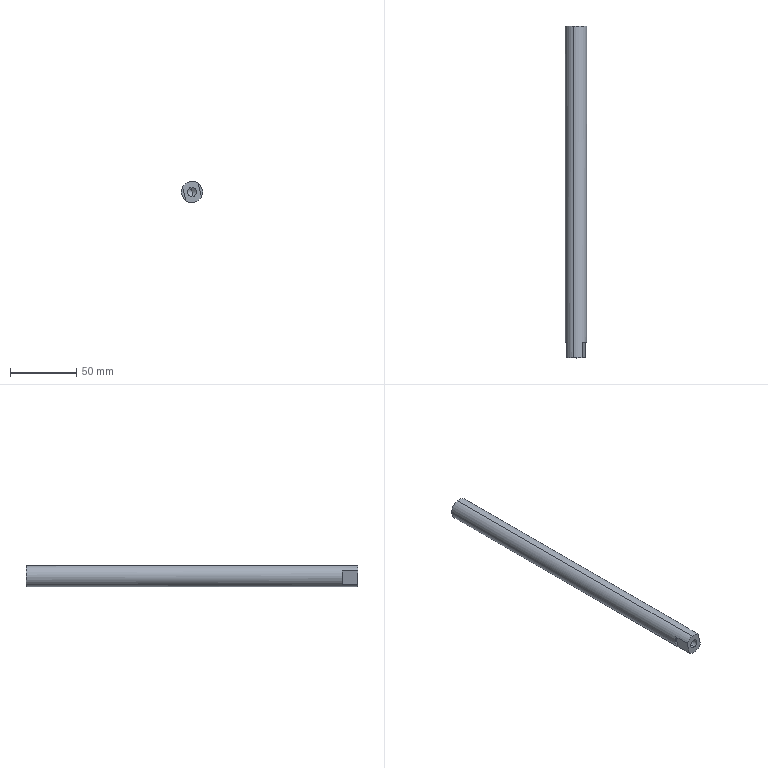Component | SolidWorks | 20-MaterialTrayLifting-1111-1_22-BF-1111-11 | 1 solid | 16 faces | box 16 x 250 x 16 mm | volume 48433 mm3 | cylinder 6 | plane 6 | cone 4 | commonest cylinder face diameters 6.8 x4 16 x2 | material 40CR
build123d program:
from build123d import *

# Parameters (mm, degrees)
SKETCH1_R             = 8
BOSS_EXTRUDE1_DEPTH   = 250
M8_TAPPED_HOLE2_D     = 6.8
M8_TAPPED_HOLE2_DEPTH = 19.75
M8_TAPPED_HOLE2_TIP   = 2.043
M8_TAPPED_HOLE3_D     = 6.8
M8_TAPPED_HOLE3_DEPTH = 19.75
M8_TAPPED_HOLE3_TIP   = 2.043
SKETCH11_W            = 23.8
SKETCH11_H            = 6.865
CUT_EXTRUDE1_DEPTH    = 12


with BuildPart() as part:
    # Sketch1 → Boss-Extrude1 (new body)
    with BuildSketch(Plane.XY):
        Circle(SKETCH1_R)
    extrude(amount=BOSS_EXTRUDE1_DEPTH)

    # M8 Tapped Hole2
    with Locations(Plane.XY.offset(250)):
        with Locations((0, 0)):
            Hole(M8_TAPPED_HOLE2_D / 2, depth=M8_TAPPED_HOLE2_DEPTH)
            with Locations((0, 0, -(M8_TAPPED_HOLE2_DEPTH + M8_TAPPED_HOLE2_TIP / 2))):  # 118° drill point
                Cone(0, M8_TAPPED_HOLE2_D / 2, M8_TAPPED_HOLE2_TIP, mode=Mode.SUBTRACT)

    # M8 Tapped Hole3
    with Locations(Plane(origin=(0, 0, 0), x_dir=(-1, 0, 0), z_dir=(0, 0, -1))):
        with Locations((0, 0)):
            Hole(M8_TAPPED_HOLE3_D / 2, depth=M8_TAPPED_HOLE3_DEPTH)
            with Locations((0, 0, -(M8_TAPPED_HOLE3_DEPTH + M8_TAPPED_HOLE3_TIP / 2))):  # 118° drill point
                Cone(0, M8_TAPPED_HOLE3_D / 2, M8_TAPPED_HOLE3_TIP, mode=Mode.SUBTRACT)

    # Sketch11 → Cut-Extrude1 (cut)
    with BuildSketch(Plane.XY.offset(250)):
        with Locations((1.299, 9.432)):
            Rectangle(SKETCH11_W, SKETCH11_H)
        with Locations((1.299, -9.432)):
            Rectangle(SKETCH11_W, SKETCH11_H)
    extrude(amount=-CUT_EXTRUDE1_DEPTH, mode=Mode.SUBTRACT)


solid = part.part

# Placed as in the assembly
solid = solid.moved(Location((68.428, 539.224, 1438.056), (90, 0, 102.883)))
STEP:
#1=CARTESIAN_POINT('',(2.724,20.452,56.486));
#2=VERTEX_POINT('',#1);
#3=CARTESIAN_POINT('',(2.664,20.452,56.747));
#4=VERTEX_POINT('',#3);
#5=CARTESIAN_POINT('',(2.694,20.452,56.616));
#6=DIRECTION('',(0.,1.,-0.));
#7=DIRECTION('',(-0.223,0.,0.9748));
#8=AXIS2_PLACEMENT_3D('',#5,#6,#7);
#9=CIRCLE('',#8,0.1339);
#10=EDGE_CURVE('',#2,#4,#9,.T.);
#11=ORIENTED_EDGE('',*,*,#10,.F.);
#12=CARTESIAN_POINT('',(2.724,21.229,56.486));
#13=VERTEX_POINT('',#12);
#14=CARTESIAN_POINT('',(2.724,21.229,56.486));
#15=DIRECTION('',(0.,1.,-0.));
#16=VECTOR('',#15,39.37);
#17=LINE('',#14,#16);
#18=EDGE_CURVE('',#2,#13,#17,.T.);
#19=ORIENTED_EDGE('',*,*,#18,.T.);
#20=CARTESIAN_POINT('',(2.664,21.229,56.747));
#21=VERTEX_POINT('',#20);
#22=CARTESIAN_POINT('',(2.694,21.229,56.616));
#23=DIRECTION('',(0.,1.,-0.));
#24=DIRECTION('',(-0.223,0.,0.9748));
#25=AXIS2_PLACEMENT_3D('',#22,#23,#24);
#26=CIRCLE('',#25,0.1339);
#27=EDGE_CURVE('',#13,#21,#26,.T.);
#28=ORIENTED_EDGE('',*,*,#27,.T.);
#29=CARTESIAN_POINT('',(2.664,21.229,56.747));
#30=DIRECTION('',(0.,1.,-0.));
#31=VECTOR('',#30,39.37);
#32=LINE('',#29,#31);
#33=EDGE_CURVE('',#4,#21,#32,.T.);
#34=ORIENTED_EDGE('',*,*,#33,.F.);
#35=EDGE_LOOP('',(#11,#19,#28,#34));
#36=FACE_OUTER_BOUND('',#35,.T.);
#37=CARTESIAN_POINT('',(2.694,21.229,56.616));
#38=DIRECTION('',(0.,1.,-0.));
#39=DIRECTION('',(-0.223,0.,0.9748));
#40=AXIS2_PLACEMENT_3D('',#37,#38,#39);
#41=CYLINDRICAL_SURFACE('',#40,0.1339);
#42=ADVANCED_FACE('',(#36),#41,.F.);
#43=CARTESIAN_POINT('',(2.694,20.371,56.616));
#44=VERTEX_POINT('',#43);
#45=CARTESIAN_POINT('',(2.664,20.452,56.747));
#46=DIRECTION('',(-0.1911,0.515,0.8356));
#47=VECTOR('',#46,39.37);
#48=LINE('',#45,#47);
#49=EDGE_CURVE('',#44,#4,#48,.T.);
#50=ORIENTED_EDGE('',*,*,#49,.F.);
#51=CARTESIAN_POINT('',(2.724,20.452,56.486));
#52=DIRECTION('',(0.1911,0.515,-0.8356));
#53=VECTOR('',#52,39.37);
#54=LINE('',#51,#53);
#55=EDGE_CURVE('',#44,#2,#54,.T.);
#56=ORIENTED_EDGE('',*,*,#55,.T.);
#57=ORIENTED_EDGE('',*,*,#10,.T.);
#58=EDGE_LOOP('',(#50,#56,#57));
#59=FACE_OUTER_BOUND('',#58,.T.);
#60=CARTESIAN_POINT('',(2.694,20.452,56.616));
#61=DIRECTION('',(0.,1.,-0.));
#62=DIRECTION('',(-0.223,0.,0.9748));
#63=AXIS2_PLACEMENT_3D('',#60,#61,#62);
#64=CONICAL_SURFACE('',#63,0.1339,1.03);
#65=ADVANCED_FACE('',(#59),#64,.F.);
#66=CARTESIAN_POINT('',(2.664,12.164,56.747));
#67=VERTEX_POINT('',#66);
#68=CARTESIAN_POINT('',(2.724,12.164,56.486));
#69=VERTEX_POINT('',#68);
#70=CARTESIAN_POINT('',(2.694,12.164,56.616));
#71=DIRECTION('',(-0.,-1.,0.));
#72=DIRECTION('',(0.223,0.,-0.9748));
#73=AXIS2_PLACEMENT_3D('',#70,#71,#72);
#74=CIRCLE('',#73,0.1339);
#75=EDGE_CURVE('',#67,#69,#74,.T.);
#76=ORIENTED_EDGE('',*,*,#75,.F.);
#77=CARTESIAN_POINT('',(2.664,11.387,56.747));
#78=VERTEX_POINT('',#77);
#79=CARTESIAN_POINT('',(2.664,11.387,56.747));
#80=DIRECTION('',(-0.,-1.,0.));
#81=VECTOR('',#80,39.37);
#82=LINE('',#79,#81);
#83=EDGE_CURVE('',#67,#78,#82,.T.);
#84=ORIENTED_EDGE('',*,*,#83,.T.);
#85=CARTESIAN_POINT('',(2.724,11.387,56.486));
#86=VERTEX_POINT('',#85);
#87=CARTESIAN_POINT('',(2.694,11.387,56.616));
#88=DIRECTION('',(-0.,-1.,0.));
#89=DIRECTION('',(0.223,0.,-0.9748));
#90=AXIS2_PLACEMENT_3D('',#87,#88,#89);
#91=CIRCLE('',#90,0.1339);
#92=EDGE_CURVE('',#78,#86,#91,.T.);
#93=ORIENTED_EDGE('',*,*,#92,.T.);
#94=CARTESIAN_POINT('',(2.724,11.387,56.486));
#95=DIRECTION('',(-0.,-1.,0.));
#96=VECTOR('',#95,39.37);
#97=LINE('',#94,#96);
#98=EDGE_CURVE('',#69,#86,#97,.T.);
#99=ORIENTED_EDGE('',*,*,#98,.F.);
#100=EDGE_LOOP('',(#76,#84,#93,#99));
#101=FACE_OUTER_BOUND('',#100,.T.);
#102=CARTESIAN_POINT('',(2.694,11.387,56.616));
#103=DIRECTION('',(-0.,-1.,0.));
#104=DIRECTION('',(0.223,0.,-0.9748));
#105=AXIS2_PLACEMENT_3D('',#102,#103,#104);
#106=CYLINDRICAL_SURFACE('',#105,0.1339);
#107=ADVANCED_FACE('',(#101),#106,.F.);
#108=CARTESIAN_POINT('',(2.694,12.245,56.616));
#109=VERTEX_POINT('',#108);
#110=CARTESIAN_POINT('',(2.724,12.164,56.486));
#111=DIRECTION('',(0.1911,-0.515,-0.8356));
#112=VECTOR('',#111,39.37);
#113=LINE('',#110,#112);
#114=EDGE_CURVE('',#109,#69,#113,.T.);
#115=ORIENTED_EDGE('',*,*,#114,.F.);
#116=CARTESIAN_POINT('',(2.664,12.164,56.747));
#117=DIRECTION('',(-0.1911,-0.515,0.8356));
#118=VECTOR('',#117,39.37);
#119=LINE('',#116,#118);
#120=EDGE_CURVE('',#109,#67,#119,.T.);
#121=ORIENTED_EDGE('',*,*,#120,.T.);
#122=ORIENTED_EDGE('',*,*,#75,.T.);
#123=EDGE_LOOP('',(#115,#121,#122));
#124=FACE_OUTER_BOUND('',#123,.T.);
#125=CARTESIAN_POINT('',(2.694,12.164,56.616));
#126=DIRECTION('',(-0.,-1.,0.));
#127=DIRECTION('',(0.223,0.,-0.9748));
#128=AXIS2_PLACEMENT_3D('',#125,#126,#127);
#129=CONICAL_SURFACE('',#128,0.1339,1.03);
#130=ADVANCED_FACE('',(#124),#129,.F.);
#131=CARTESIAN_POINT('',(2.764,11.387,56.309));
#132=VERTEX_POINT('',#131);
#133=CARTESIAN_POINT('',(2.971,11.387,56.466));
#134=VERTEX_POINT('',#133);
#135=CARTESIAN_POINT('',(2.694,11.387,56.616));
#136=DIRECTION('',(-0.,-1.,0.));
#137=DIRECTION('',(0.223,0.,-0.9748));
#138=AXIS2_PLACEMENT_3D('',#135,#136,#137);
#139=CIRCLE('',#138,0.315);
#140=EDGE_CURVE('',#132,#134,#139,.T.);
#141=ORIENTED_EDGE('',*,*,#140,.F.);
#142=CARTESIAN_POINT('',(2.764,21.229,56.309));
#143=VERTEX_POINT('',#142);
#144=CARTESIAN_POINT('',(2.764,11.387,56.309));
#145=DIRECTION('',(0.,1.,-0.));
#146=VECTOR('',#145,39.37);
#147=LINE('',#144,#146);
#148=EDGE_CURVE('',#132,#143,#147,.T.);
#149=ORIENTED_EDGE('',*,*,#148,.T.);
#150=CARTESIAN_POINT('',(2.624,21.229,56.923));
#151=VERTEX_POINT('',#150);
#152=CARTESIAN_POINT('',(2.694,21.229,56.616));
#153=DIRECTION('',(-0.,-1.,0.));
#154=DIRECTION('',(0.223,0.,-0.9748));
#155=AXIS2_PLACEMENT_3D('',#152,#153,#154);
#156=CIRCLE('',#155,0.315);
#157=EDGE_CURVE('',#143,#151,#156,.T.);
#158=ORIENTED_EDGE('',*,*,#157,.T.);
#159=CARTESIAN_POINT('',(2.624,11.387,56.923));
#160=VERTEX_POINT('',#159);
#161=CARTESIAN_POINT('',(2.624,11.387,56.923));
#162=DIRECTION('',(0.,1.,-0.));
#163=VECTOR('',#162,39.37);
#164=LINE('',#161,#163);
#165=EDGE_CURVE('',#160,#151,#164,.T.);
#166=ORIENTED_EDGE('',*,*,#165,.F.);
#167=CARTESIAN_POINT('',(2.878,11.387,56.872));
#168=VERTEX_POINT('',#167);
#169=CARTESIAN_POINT('',(2.694,11.387,56.616));
#170=DIRECTION('',(-0.,-1.,0.));
#171=DIRECTION('',(0.223,0.,-0.9748));
#172=AXIS2_PLACEMENT_3D('',#169,#170,#171);
#173=CIRCLE('',#172,0.315);
#174=EDGE_CURVE('',#168,#160,#173,.T.);
#175=ORIENTED_EDGE('',*,*,#174,.F.);
#176=CARTESIAN_POINT('',(2.878,11.859,56.872));
#177=VERTEX_POINT('',#176);
#178=CARTESIAN_POINT('',(2.878,11.387,56.872));
#179=DIRECTION('',(0.,1.,-0.));
#180=VECTOR('',#179,39.37);
#181=LINE('',#178,#180);
#182=EDGE_CURVE('',#168,#177,#181,.T.);
#183=ORIENTED_EDGE('',*,*,#182,.T.);
#184=CARTESIAN_POINT('',(2.971,11.859,56.466));
#185=VERTEX_POINT('',#184);
#186=CARTESIAN_POINT('',(2.694,11.859,56.616));
#187=DIRECTION('',(-0.,-1.,0.));
#188=DIRECTION('',(0.223,0.,-0.9748));
#189=AXIS2_PLACEMENT_3D('',#186,#187,#188);
#190=CIRCLE('',#189,0.315);
#191=EDGE_CURVE('',#185,#177,#190,.T.);
#192=ORIENTED_EDGE('',*,*,#191,.F.);
#193=CARTESIAN_POINT('',(2.971,11.387,56.466));
#194=DIRECTION('',(-0.,-1.,0.));
#195=VECTOR('',#194,39.37);
#196=LINE('',#193,#195);
#197=EDGE_CURVE('',#185,#134,#196,.T.);
#198=ORIENTED_EDGE('',*,*,#197,.T.);
#199=EDGE_LOOP('',(#141,#149,#158,#166,#175,#183,#192,#198));
#200=FACE_OUTER_BOUND('',#199,.T.);
#201=CARTESIAN_POINT('',(2.694,11.387,56.616));
#202=DIRECTION('',(0.,1.,-0.));
#203=DIRECTION('',(-0.223,0.,0.9748));
#204=AXIS2_PLACEMENT_3D('',#201,#202,#203);
#205=CYLINDRICAL_SURFACE('',#204,0.315);
#206=ADVANCED_FACE('',(#200),#205,.T.);
#207=ORIENTED_EDGE('',*,*,#148,.F.);
#208=CARTESIAN_POINT('',(2.51,11.387,56.361));
#209=VERTEX_POINT('',#208);
#210=CARTESIAN_POINT('',(2.694,11.387,56.616));
#211=DIRECTION('',(-0.,-1.,0.));
#212=DIRECTION('',(0.223,0.,-0.9748));
#213=AXIS2_PLACEMENT_3D('',#210,#211,#212);
#214=CIRCLE('',#213,0.315);
#215=EDGE_CURVE('',#209,#132,#214,.T.);
#216=ORIENTED_EDGE('',*,*,#215,.F.);
#217=CARTESIAN_POINT('',(2.51,11.859,56.361));
#218=VERTEX_POINT('',#217);
#219=CARTESIAN_POINT('',(2.51,11.387,56.361));
#220=DIRECTION('',(0.,1.,-0.));
#221=VECTOR('',#220,39.37);
#222=LINE('',#219,#221);
#223=EDGE_CURVE('',#209,#218,#222,.T.);
#224=ORIENTED_EDGE('',*,*,#223,.T.);
#225=CARTESIAN_POINT('',(2.417,11.859,56.767));
#226=VERTEX_POINT('',#225);
#227=CARTESIAN_POINT('',(2.694,11.859,56.616));
#228=DIRECTION('',(0.,1.,-0.));
#229=DIRECTION('',(-0.223,0.,0.9748));
#230=AXIS2_PLACEMENT_3D('',#227,#228,#229);
#231=CIRCLE('',#230,0.315);
#232=EDGE_CURVE('',#218,#226,#231,.T.);
#233=ORIENTED_EDGE('',*,*,#232,.T.);
#234=CARTESIAN_POINT('',(2.417,11.387,56.767));
#235=VERTEX_POINT('',#234);
#236=CARTESIAN_POINT('',(2.417,11.387,56.767));
#237=DIRECTION('',(-0.,-1.,0.));
#238=VECTOR('',#237,39.37);
#239=LINE('',#236,#238);
#240=EDGE_CURVE('',#226,#235,#239,.T.);
#241=ORIENTED_EDGE('',*,*,#240,.T.);
#242=CARTESIAN_POINT('',(2.694,11.387,56.616));
#243=DIRECTION('',(-0.,-1.,0.));
#244=DIRECTION('',(0.223,0.,-0.9748));
#245=AXIS2_PLACEMENT_3D('',#242,#243,#244);
#246=CIRCLE('',#245,0.315);
#247=EDGE_CURVE('',#160,#235,#246,.T.);
#248=ORIENTED_EDGE('',*,*,#247,.F.);
#249=ORIENTED_EDGE('',*,*,#165,.T.);
#250=CARTESIAN_POINT('',(2.694,21.229,56.616));
#251=DIRECTION('',(-0.,-1.,0.));
#252=DIRECTION('',(0.223,0.,-0.9748));
#253=AXIS2_PLACEMENT_3D('',#250,#251,#252);
#254=CIRCLE('',#253,0.315);
#255=EDGE_CURVE('',#151,#143,#254,.T.);
#256=ORIENTED_EDGE('',*,*,#255,.T.);
#257=EDGE_LOOP('',(#207,#216,#224,#233,#241,#248,#249,#256));
#258=FACE_OUTER_BOUND('',#257,.T.);
#259=CARTESIAN_POINT('',(2.694,11.387,56.616));
#260=DIRECTION('',(0.,1.,-0.));
#261=DIRECTION('',(-0.223,0.,0.9748));
#262=AXIS2_PLACEMENT_3D('',#259,#260,#261);
#263=CYLINDRICAL_SURFACE('',#262,0.315);
#264=ADVANCED_FACE('',(#258),#263,.T.);
#265=CARTESIAN_POINT('',(2.464,11.387,56.564));
#266=DIRECTION('',(-0.223,0.,0.9748));
#267=VECTOR('',#266,39.37);
#268=LINE('',#265,#267);
#269=EDGE_CURVE('',#209,#235,#268,.T.);
#270=ORIENTED_EDGE('',*,*,#269,.F.);
#271=ORIENTED_EDGE('',*,*,#215,.T.);
#272=ORIENTED_EDGE('',*,*,#140,.T.);
#273=CARTESIAN_POINT('',(2.924,11.387,56.669));
#274=DIRECTION('',(0.223,-0.,-0.9748));
#275=VECTOR('',#274,39.37);
#276=LINE('',#273,#275);
#277=EDGE_CURVE('',#168,#134,#276,.T.);
#278=ORIENTED_EDGE('',*,*,#277,.F.);
#279=ORIENTED_EDGE('',*,*,#174,.T.);
#280=ORIENTED_EDGE('',*,*,#247,.T.);
#281=EDGE_LOOP('',(#270,#271,#272,#278,#279,#280));
#282=FACE_OUTER_BOUND('',#281,.T.);
#283=CARTESIAN_POINT('',(2.694,11.387,56.616));
#284=DIRECTION('',(-0.,-1.,0.));
#285=DIRECTION('',(0.223,0.,-0.9748));
#286=AXIS2_PLACEMENT_3D('',#283,#284,#285);
#287=CIRCLE('',#286,0.1339);
#288=EDGE_CURVE('',#86,#78,#287,.T.);
#289=ORIENTED_EDGE('',*,*,#288,.F.);
#290=ORIENTED_EDGE('',*,*,#92,.F.);
#291=EDGE_LOOP('',(#289,#290));
#292=FACE_BOUND('',#291,.T.);
#293=CARTESIAN_POINT('',(2.694,11.387,56.616));
#294=DIRECTION('',(-0.,-1.,0.));
#295=DIRECTION('',(0.223,-0.,-0.9748));
#296=AXIS2_PLACEMENT_3D('',#293,#294,#295);
#297=PLANE('',#296);
#298=ADVANCED_FACE('',(#282,#292),#297,.T.);
#299=CARTESIAN_POINT('',(2.694,21.229,56.616));
#300=DIRECTION('',(0.,1.,-0.));
#301=DIRECTION('',(-0.223,0.,0.9748));
#302=AXIS2_PLACEMENT_3D('',#299,#300,#301);
#303=CIRCLE('',#302,0.1339);
#304=EDGE_CURVE('',#21,#13,#303,.T.);
#305=ORIENTED_EDGE('',*,*,#304,.F.);
#306=ORIENTED_EDGE('',*,*,#27,.F.);
#307=EDGE_LOOP('',(#305,#306));
#308=FACE_BOUND('',#307,.T.);
#309=ORIENTED_EDGE('',*,*,#255,.F.);
#310=ORIENTED_EDGE('',*,*,#157,.F.);
#311=EDGE_LOOP('',(#309,#310));
#312=FACE_OUTER_BOUND('',#311,.T.);
#313=CARTESIAN_POINT('',(2.694,21.229,56.616));
#314=DIRECTION('',(-0.,-1.,0.));
#315=DIRECTION('',(0.223,-0.,-0.9748));
#316=AXIS2_PLACEMENT_3D('',#313,#314,#315);
#317=PLANE('',#316);
#318=ADVANCED_FACE('',(#308,#312),#317,.F.);
#319=ORIENTED_EDGE('',*,*,#120,.F.);
#320=ORIENTED_EDGE('',*,*,#114,.T.);
#321=CARTESIAN_POINT('',(2.694,12.164,56.616));
#322=DIRECTION('',(-0.,-1.,0.));
#323=DIRECTION('',(0.223,0.,-0.9748));
#324=AXIS2_PLACEMENT_3D('',#321,#322,#323);
#325=CIRCLE('',#324,0.1339);
#326=EDGE_CURVE('',#69,#67,#325,.T.);
#327=ORIENTED_EDGE('',*,*,#326,.T.);
#328=EDGE_LOOP('',(#319,#320,#327));
#329=FACE_OUTER_BOUND('',#328,.T.);
#330=CARTESIAN_POINT('',(2.694,12.164,56.616));
#331=DIRECTION('',(-0.,-1.,0.));
#332=DIRECTION('',(0.223,0.,-0.9748));
#333=AXIS2_PLACEMENT_3D('',#330,#331,#332);
#334=CONICAL_SURFACE('',#333,0.1339,1.03);
#335=ADVANCED_FACE('',(#329),#334,.F.);
#336=ORIENTED_EDGE('',*,*,#83,.F.);
#337=ORIENTED_EDGE('',*,*,#326,.F.);
#338=ORIENTED_EDGE('',*,*,#98,.T.);
#339=ORIENTED_EDGE('',*,*,#288,.T.);
#340=EDGE_LOOP('',(#336,#337,#338,#339));
#341=FACE_OUTER_BOUND('',#340,.T.);
#342=CARTESIAN_POINT('',(2.694,11.387,56.616));
#343=DIRECTION('',(-0.,-1.,0.));
#344=DIRECTION('',(0.223,0.,-0.9748));
#345=AXIS2_PLACEMENT_3D('',#342,#343,#344);
#346=CYLINDRICAL_SURFACE('',#345,0.1339);
#347=ADVANCED_FACE('',(#341),#346,.F.);
#348=ORIENTED_EDGE('',*,*,#55,.F.);
#349=ORIENTED_EDGE('',*,*,#49,.T.);
#350=CARTESIAN_POINT('',(2.694,20.452,56.616));
#351=DIRECTION('',(0.,1.,-0.));
#352=DIRECTION('',(-0.223,0.,0.9748));
#353=AXIS2_PLACEMENT_3D('',#350,#351,#352);
#354=CIRCLE('',#353,0.1339);
#355=EDGE_CURVE('',#4,#2,#354,.T.);
#356=ORIENTED_EDGE('',*,*,#355,.T.);
#357=EDGE_LOOP('',(#348,#349,#356));
#358=FACE_OUTER_BOUND('',#357,.T.);
#359=CARTESIAN_POINT('',(2.694,20.452,56.616));
#360=DIRECTION('',(0.,1.,-0.));
#361=DIRECTION('',(-0.223,0.,0.9748));
#362=AXIS2_PLACEMENT_3D('',#359,#360,#361);
#363=CONICAL_SURFACE('',#362,0.1339,1.03);
#364=ADVANCED_FACE('',(#358),#363,.F.);
#365=ORIENTED_EDGE('',*,*,#18,.F.);
#366=ORIENTED_EDGE('',*,*,#355,.F.);
#367=ORIENTED_EDGE('',*,*,#33,.T.);
#368=ORIENTED_EDGE('',*,*,#304,.T.);
#369=EDGE_LOOP('',(#365,#366,#367,#368));
#370=FACE_OUTER_BOUND('',#369,.T.);
#371=CARTESIAN_POINT('',(2.694,21.229,56.616));
#372=DIRECTION('',(0.,1.,-0.));
#373=DIRECTION('',(-0.223,0.,0.9748));
#374=AXIS2_PLACEMENT_3D('',#371,#372,#373);
#375=CYLINDRICAL_SURFACE('',#374,0.1339);
#376=ADVANCED_FACE('',(#370),#375,.F.);
#377=ORIENTED_EDGE('',*,*,#191,.T.);
#378=CARTESIAN_POINT('',(2.831,11.859,57.076));
#379=DIRECTION('',(0.223,-0.,-0.9748));
#380=VECTOR('',#379,39.37);
#381=LINE('',#378,#380);
#382=EDGE_CURVE('',#177,#185,#381,.T.);
#383=ORIENTED_EDGE('',*,*,#382,.T.);
#384=EDGE_LOOP('',(#377,#383));
#385=FACE_OUTER_BOUND('',#384,.T.);
#386=CARTESIAN_POINT('',(2.694,11.859,56.616));
#387=DIRECTION('',(-0.,-1.,0.));
#388=DIRECTION('',(0.223,-0.,-0.9748));
#389=AXIS2_PLACEMENT_3D('',#386,#387,#388);
#390=PLANE('',#389);
#391=ADVANCED_FACE('',(#385),#390,.T.);
#392=ORIENTED_EDGE('',*,*,#277,.T.);
#393=ORIENTED_EDGE('',*,*,#197,.F.);
#394=ORIENTED_EDGE('',*,*,#382,.F.);
#395=ORIENTED_EDGE('',*,*,#182,.F.);
#396=EDGE_LOOP('',(#392,#393,#394,#395));
#397=FACE_OUTER_BOUND('',#396,.T.);
#398=CARTESIAN_POINT('',(2.831,11.859,57.076));
#399=DIRECTION('',(-0.9748,0.,-0.223));
#400=DIRECTION('',(0.,1.,-0.));
#401=AXIS2_PLACEMENT_3D('',#398,#399,#400);
#402=PLANE('',#401);
#403=ADVANCED_FACE('',(#397),#402,.F.);
#404=CARTESIAN_POINT('',(2.371,11.859,56.971));
#405=DIRECTION('',(-0.223,0.,0.9748));
#406=VECTOR('',#405,39.37);
#407=LINE('',#404,#406);
#408=EDGE_CURVE('',#218,#226,#407,.T.);
#409=ORIENTED_EDGE('',*,*,#408,.T.);
#410=ORIENTED_EDGE('',*,*,#232,.F.);
#411=EDGE_LOOP('',(#409,#410));
#412=FACE_OUTER_BOUND('',#411,.T.);
#413=CARTESIAN_POINT('',(2.694,11.859,56.616));
#414=DIRECTION('',(0.,1.,-0.));
#415=DIRECTION('',(-0.223,0.,0.9748));
#416=AXIS2_PLACEMENT_3D('',#413,#414,#415);
#417=PLANE('',#416);
#418=ADVANCED_FACE('',(#412),#417,.F.);
#419=ORIENTED_EDGE('',*,*,#269,.T.);
#420=ORIENTED_EDGE('',*,*,#240,.F.);
#421=ORIENTED_EDGE('',*,*,#408,.F.);
#422=ORIENTED_EDGE('',*,*,#223,.F.);
#423=EDGE_LOOP('',(#419,#420,#421,#422));
#424=FACE_OUTER_BOUND('',#423,.T.);
#425=CARTESIAN_POINT('',(2.371,11.859,56.971));
#426=DIRECTION('',(0.9748,-0.,0.223));
#427=DIRECTION('',(-0.,-1.,0.));
#428=AXIS2_PLACEMENT_3D('',#425,#426,#427);
#429=PLANE('',#428);
#430=ADVANCED_FACE('',(#424),#429,.F.);
#431=CLOSED_SHELL('',(#42,#65,#107,#130,#206,#264,#298,#318,#335,#347,#364,#376,#391,#403,#418,#430));
#432=MANIFOLD_SOLID_BREP('',#431);
#433=CARTESIAN_POINT('',(0.,0.,0.));
#434=DIRECTION('',(0.,0.,1.));
#435=DIRECTION('',(1.,0.,0.));
#436=AXIS2_PLACEMENT_3D('',#433,#434,#435);
#437=(LENGTH_UNIT()NAMED_UNIT(*)SI_UNIT($,.METRE.));
#438=LENGTH_MEASURE_WITH_UNIT(LENGTH_MEASURE(0.0254),#437);
#439=DIMENSIONAL_EXPONENTS(1.,0.,0.,0.,0.,0.,0.);
#440=(CONVERSION_BASED_UNIT('',#438)LENGTH_UNIT()NAMED_UNIT(#439));
#441=UNCERTAINTY_MEASURE_WITH_UNIT(LENGTH_MEASURE(0.00001),#440,'','');
#442=(NAMED_UNIT(*)PLANE_ANGLE_UNIT()SI_UNIT($,.RADIAN.));
#443=(NAMED_UNIT(*)SI_UNIT($,.STERADIAN.)SOLID_ANGLE_UNIT());
#444=(GEOMETRIC_REPRESENTATION_CONTEXT(3)GLOBAL_UNCERTAINTY_ASSIGNED_CONTEXT((#441))GLOBAL_UNIT_ASSIGNED_CONTEXT((#440,#442,#443))REPRESENTATION_CONTEXT('',''));
#445=ADVANCED_BREP_SHAPE_REPRESENTATION('',(#432,#436),#444);
#446=COLOUR_RGB('',0.7922,0.8196,0.9333);
#447=FILL_AREA_STYLE_COLOUR('',#446);
#448=FILL_AREA_STYLE('',(#447));
#449=SURFACE_STYLE_FILL_AREA(#448);
#450=SURFACE_SIDE_STYLE('',(#449));
#451=SURFACE_STYLE_USAGE(.BOTH.,#450);
#452=PRESENTATION_STYLE_ASSIGNMENT((#451));
#453=STYLED_ITEM('',(#452),#432);
#454=(LENGTH_UNIT()NAMED_UNIT(*)SI_UNIT($,.METRE.));
#455=LENGTH_MEASURE_WITH_UNIT(LENGTH_MEASURE(0.0254),#454);
#456=DIMENSIONAL_EXPONENTS(1.,0.,0.,0.,0.,0.,0.);
#457=(CONVERSION_BASED_UNIT('',#455)LENGTH_UNIT()NAMED_UNIT(#456));
#458=UNCERTAINTY_MEASURE_WITH_UNIT(LENGTH_MEASURE(0.00001),#457,'','');
#459=(NAMED_UNIT(*)PLANE_ANGLE_UNIT()SI_UNIT($,.RADIAN.));
#460=(NAMED_UNIT(*)SI_UNIT($,.STERADIAN.)SOLID_ANGLE_UNIT());
#461=(GEOMETRIC_REPRESENTATION_CONTEXT(3)GLOBAL_UNCERTAINTY_ASSIGNED_CONTEXT((#458))GLOBAL_UNIT_ASSIGNED_CONTEXT((#457,#459,#460))REPRESENTATION_CONTEXT('',''));
#462=MECHANICAL_DESIGN_GEOMETRIC_PRESENTATION_REPRESENTATION('',(#453),#461);
#463=PRESENTATION_LAYER_ASSIGNMENT('','',(#453));